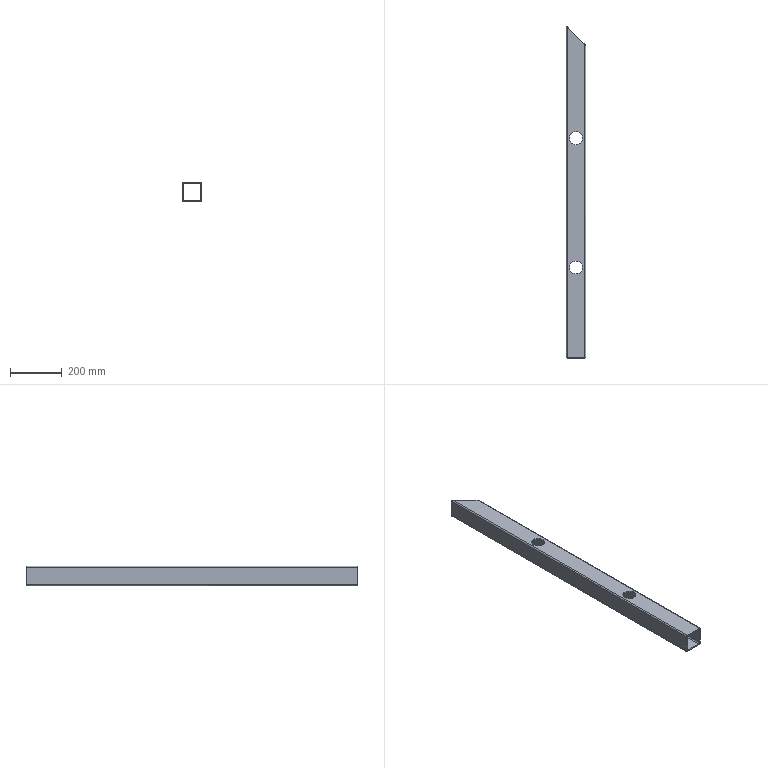Component | NX | VERTICAL_BRACKET_UPRIGHT_BEAM_2 | 1 solid | 22 faces | volume 1407848 mm3 | cylinder 12 | plane 10 | commonest cylinder face diameters 8 x8 50 x4